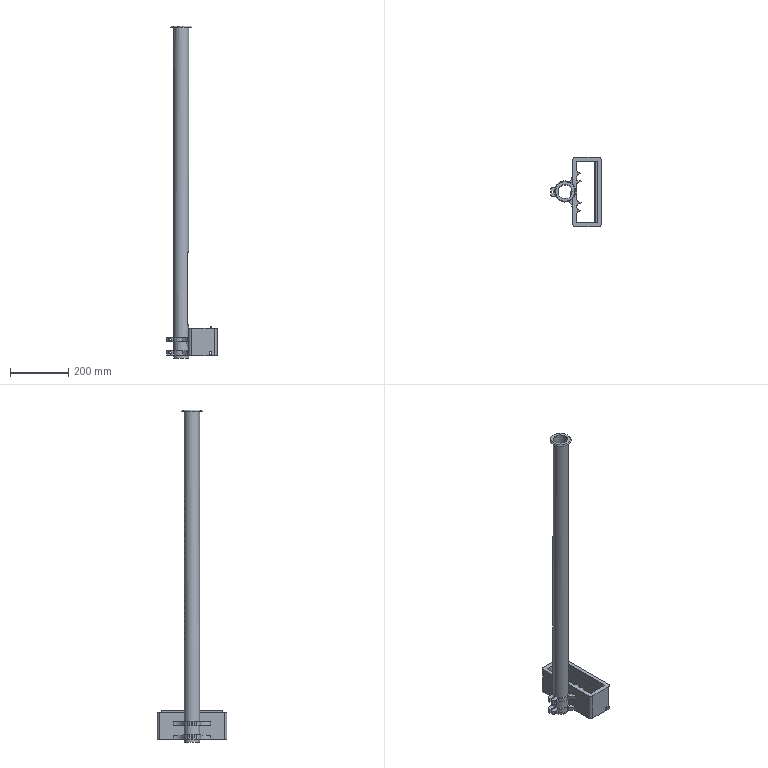Component | NX | MODEL4 | 1 solid | 100 faces | volume 1232489 mm3 | plane 65 | cylinder 34 | cone 1 | commonest cylinder face diameters 20 x11 59.673 x4 8 x4 12 x4 80 x4 30 x2 10 x2 52 x1